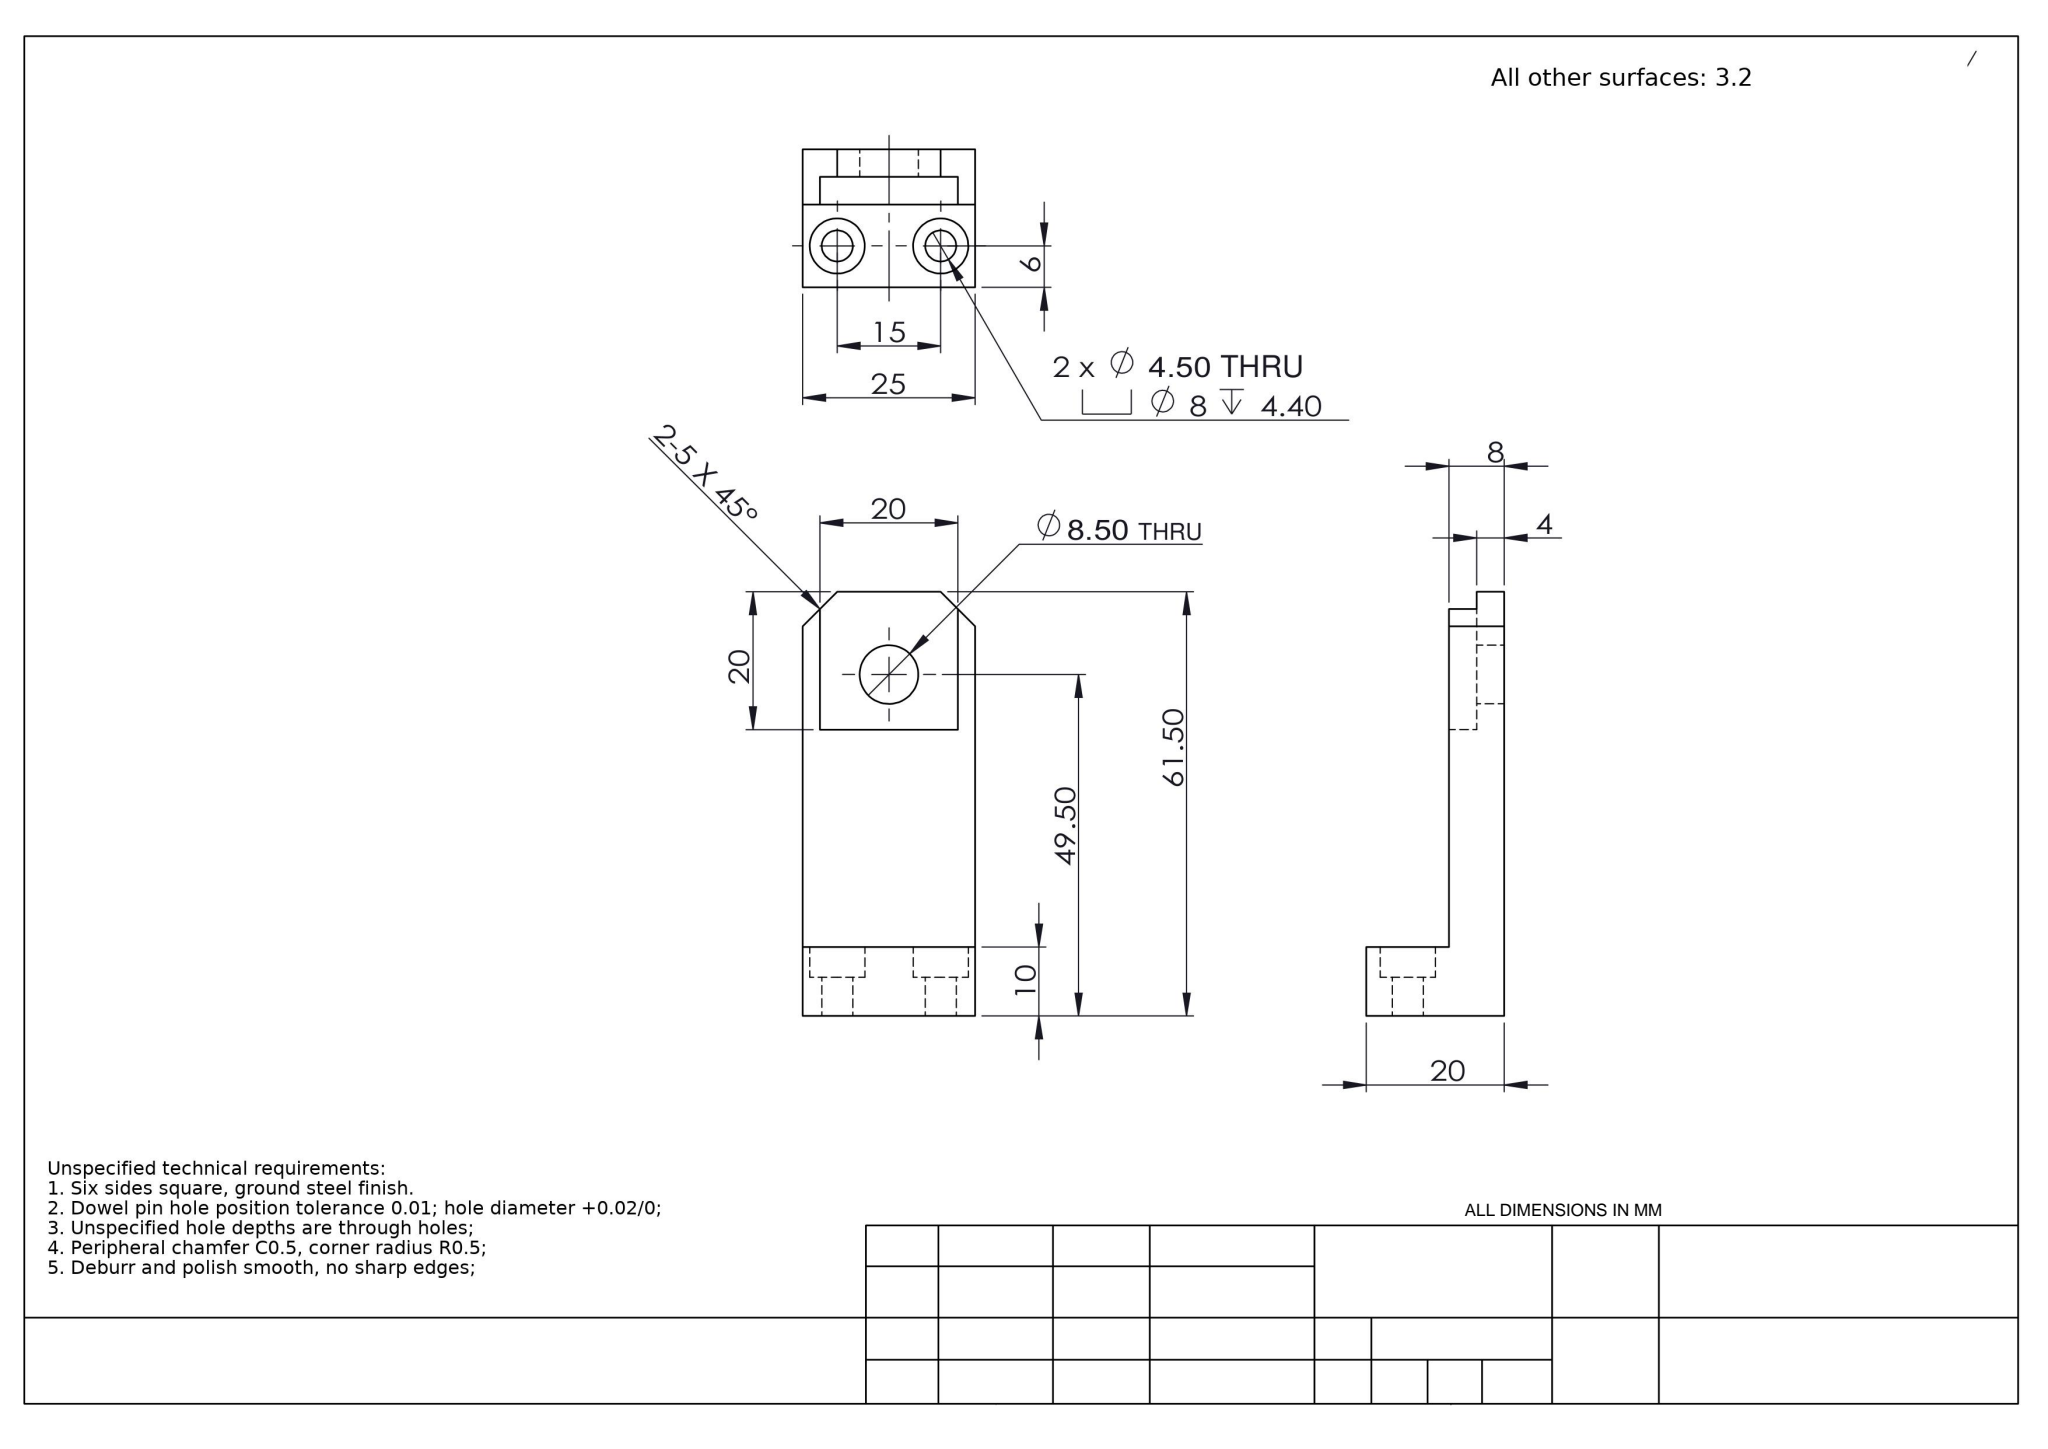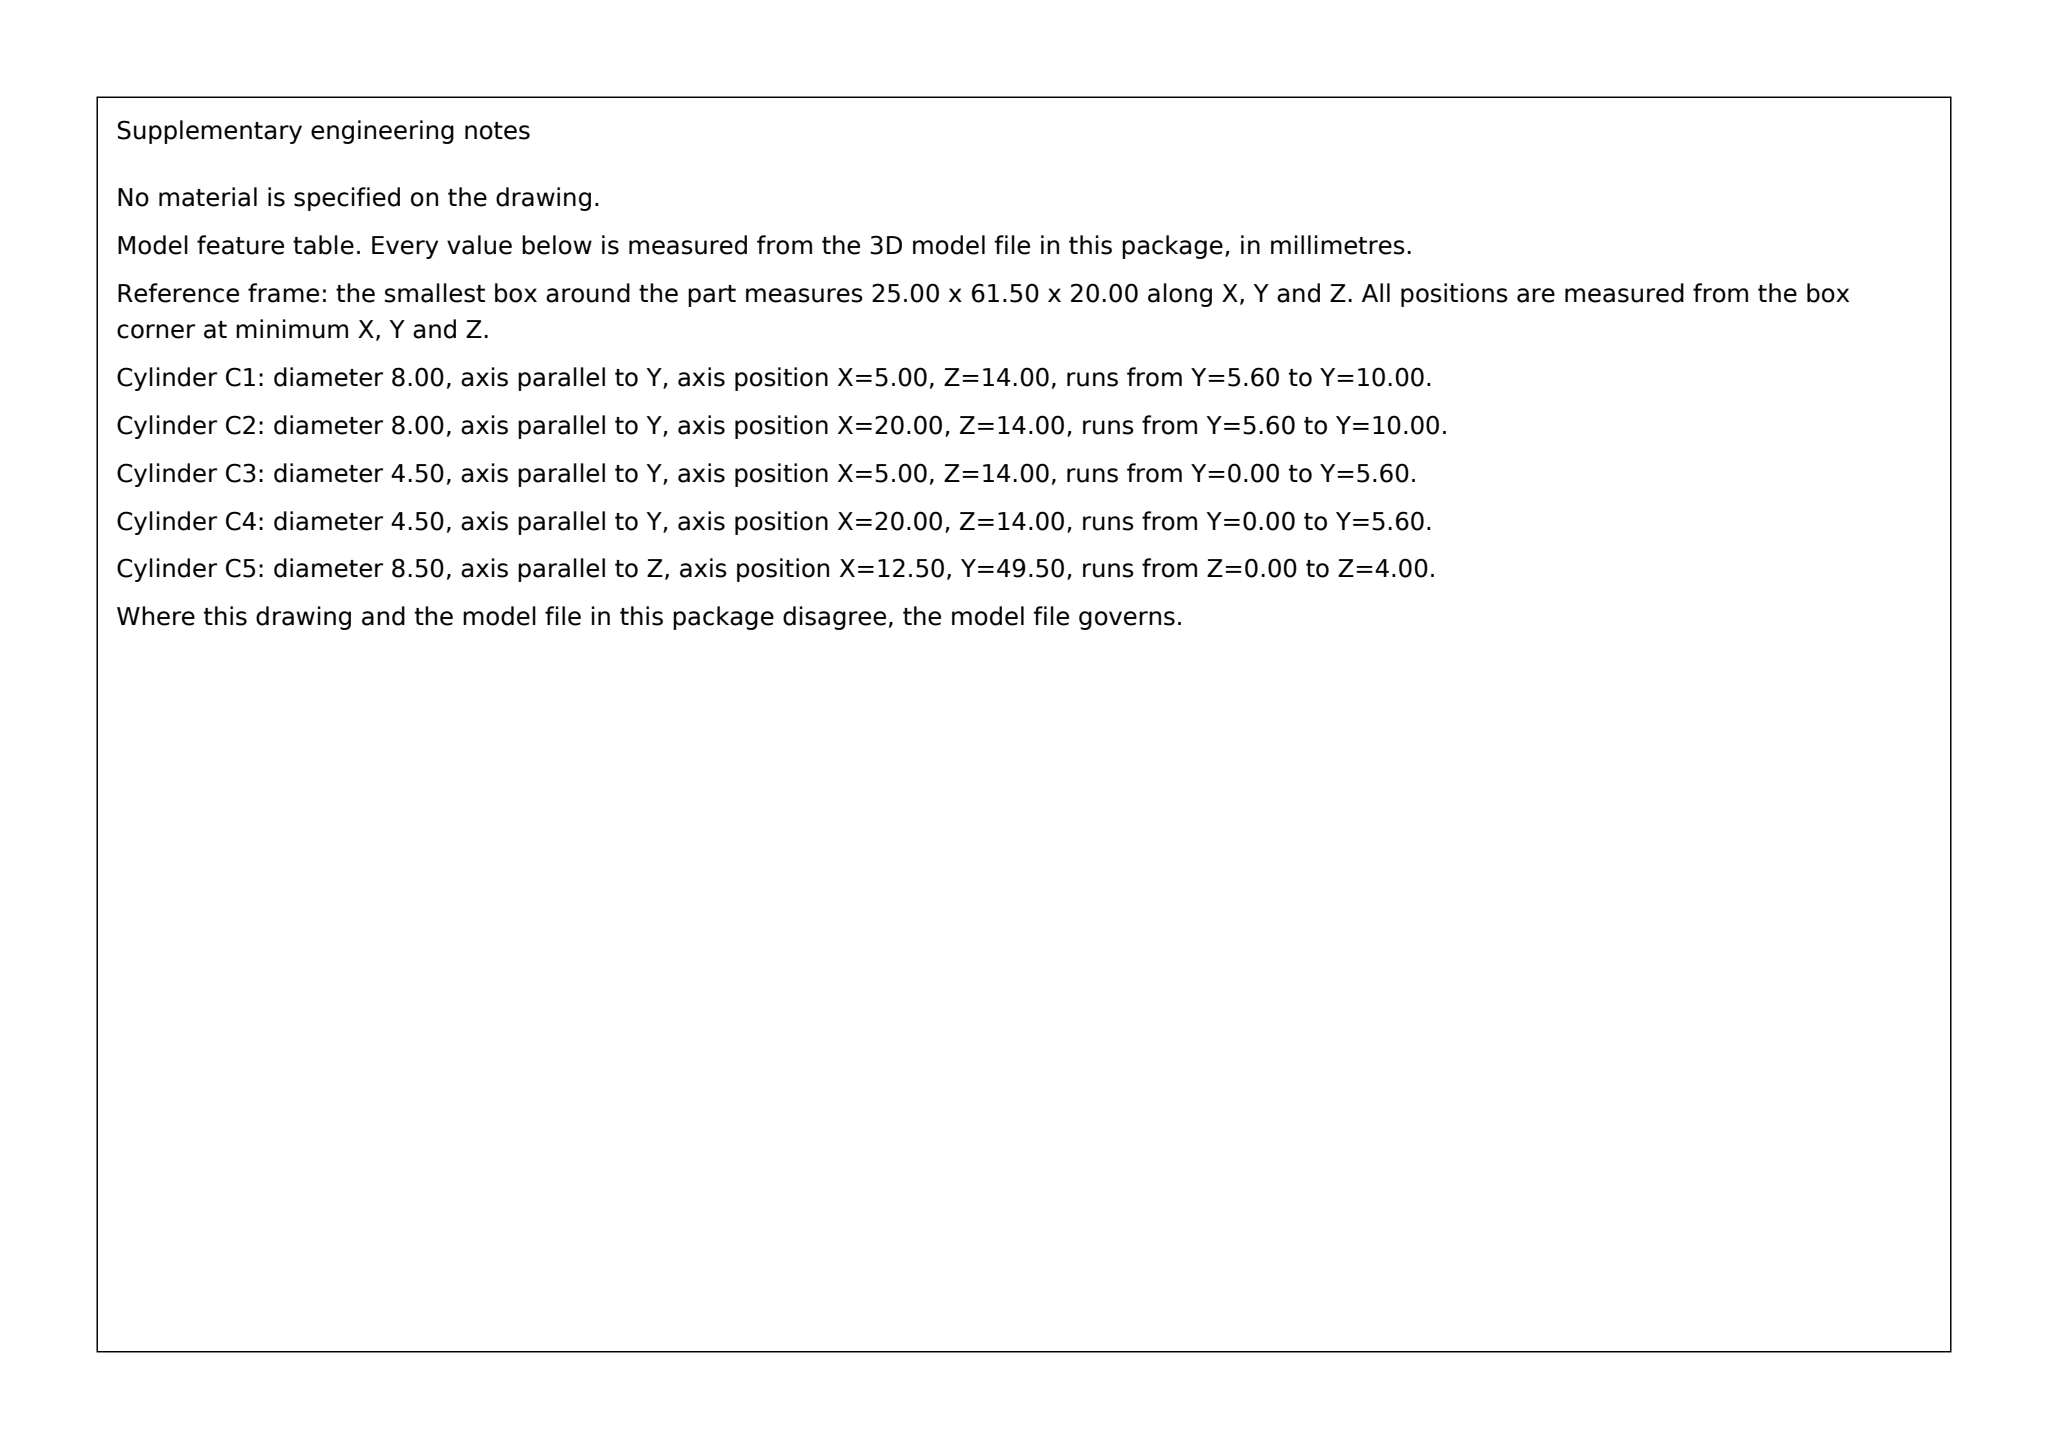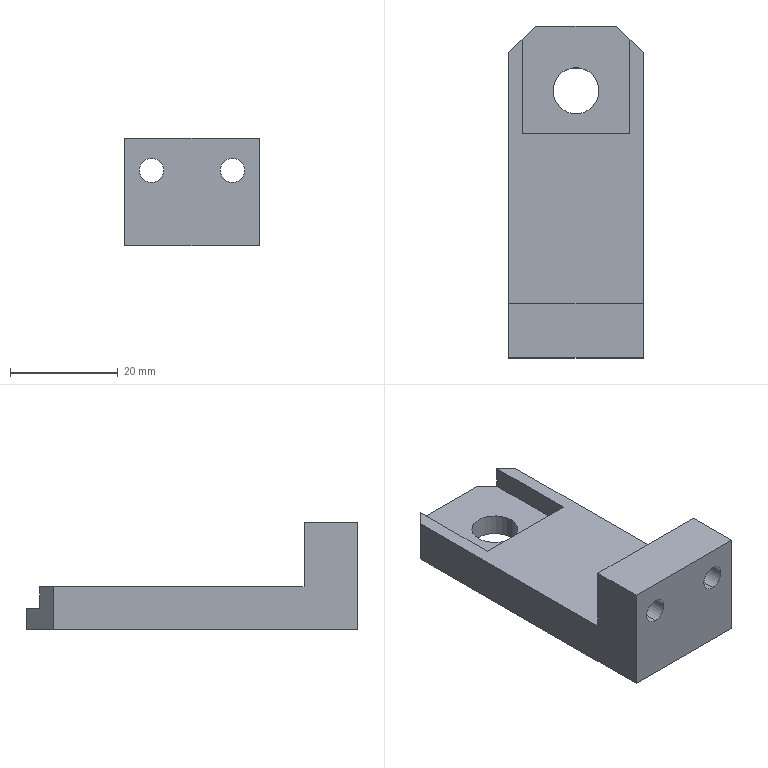Part | SolidWorks | mm | material 6060-T6 | 1 solid | 26 faces | box 25 x 61.5 x 20 mm | volume 12678 mm3 | plane 16 | cylinder 10 | commonest cylinder face diameters 8 x4 4.5 x4 8.5 x2
build123d program:
from build123d import *

# Parameters (mm, degrees)
SKETCH1_W                                       = 25
SKETCH1_H                                       = 20
BOSS_EXTRUDE1_DEPTH                             = 61.5
SKETCH2_W                                       = 12
SKETCH2_H                                       = 51.5
CUT_EXTRUDE1_DEPTH                              = 68.136
SKETCH3_R                                       = 4.25
CUT_EXTRUDE2_DEPTH                              = 64.894
M4_HEX_SOCKET_HEAD_CAP_SCREW_CBORE1_D           = 4.5
M4_HEX_SOCKET_HEAD_CAP_SCREW_CBORE1_CBORE_D     = 8
M4_HEX_SOCKET_HEAD_CAP_SCREW_CBORE1_CBORE_DEPTH = 4.4
CHAMFER1_SIZE                                   = 5
SKETCH7_W                                       = 20
SKETCH7_H                                       = 20
CUT_EXTRUDE3_DEPTH                              = 4


with BuildPart() as part:
    # Sketch1 → Boss-Extrude1 (new body)
    with BuildSketch(Plane(origin=(0, 0, 0), x_dir=(1, 0, 0), z_dir=(0, 1, 0))):
        Rectangle(SKETCH1_W, SKETCH1_H)
    extrude(amount=BOSS_EXTRUDE1_DEPTH)

    # Sketch2 → Cut-Extrude1 (cut, through all)
    with BuildSketch(Plane(origin=(12.5, 0, 0), x_dir=(0, 0, -1), z_dir=(1, 0, 0))):
        with Locations((-4, 35.75)):
            Rectangle(SKETCH2_W, SKETCH2_H)
    extrude(amount=-CUT_EXTRUDE1_DEPTH, mode=Mode.SUBTRACT)

    # Sketch3 → Cut-Extrude2 (cut, through all)
    with BuildSketch(Plane.XY.offset(-2)):
        with Locations((0, 49.5)):
            Circle(SKETCH3_R)
    extrude(amount=-CUT_EXTRUDE2_DEPTH, mode=Mode.SUBTRACT)

    # M4 Hex Socket Head Cap Screw CBORE1 (through all)
    with Locations(Plane(origin=(0, 10, 0), x_dir=(1, 0, 0), z_dir=(0, 1, 0))):
        with Locations((-7.5, -4), (7.5, -4)):
            CounterBoreHole(M4_HEX_SOCKET_HEAD_CAP_SCREW_CBORE1_D / 2, M4_HEX_SOCKET_HEAD_CAP_SCREW_CBORE1_CBORE_D / 2, M4_HEX_SOCKET_HEAD_CAP_SCREW_CBORE1_CBORE_DEPTH)

    # Chamfer1
    chamfer1_edges = [part.edges().sort_by_distance(p)[0] for p in [
        (-12.5, 61.5, -6),
        (12.5, 61.5, -6),
    ]]
    chamfer(chamfer1_edges, length=CHAMFER1_SIZE)

    # Sketch7 → Cut-Extrude3 (cut)
    with BuildSketch(Plane.XY.offset(-2)):
        with Locations((0, 51.5)):
            Rectangle(SKETCH7_W, SKETCH7_H)
    extrude(amount=-CUT_EXTRUDE3_DEPTH, mode=Mode.SUBTRACT)


solid = part.part
STEP:
#1=CARTESIAN_POINT('',(-7.5,5.6,-0.));
#2=VERTEX_POINT('',#1);
#3=CARTESIAN_POINT('',(-7.5,5.6,8.));
#4=VERTEX_POINT('',#3);
#5=CARTESIAN_POINT('',(-7.5,5.6,4.));
#6=DIRECTION('',(0.,1.,0.));
#7=DIRECTION('',(0.,0.,1.));
#8=AXIS2_PLACEMENT_3D('',#5,#6,#7);
#9=CIRCLE('',#8,4.);
#10=EDGE_CURVE('',#2,#4,#9,.T.);
#11=ORIENTED_EDGE('',*,*,#10,.F.);
#12=CARTESIAN_POINT('',(-7.5,10.,-0.));
#13=VERTEX_POINT('',#12);
#14=CARTESIAN_POINT('',(-7.5,10.,-0.));
#15=DIRECTION('',(0.,1.,0.));
#16=VECTOR('',#15,1000.);
#17=LINE('',#14,#16);
#18=EDGE_CURVE('',#2,#13,#17,.T.);
#19=ORIENTED_EDGE('',*,*,#18,.T.);
#20=CARTESIAN_POINT('',(-7.5,10.,8.));
#21=VERTEX_POINT('',#20);
#22=CARTESIAN_POINT('',(-7.5,10.,4.));
#23=DIRECTION('',(0.,1.,0.));
#24=DIRECTION('',(0.,0.,1.));
#25=AXIS2_PLACEMENT_3D('',#22,#23,#24);
#26=CIRCLE('',#25,4.);
#27=EDGE_CURVE('',#13,#21,#26,.T.);
#28=ORIENTED_EDGE('',*,*,#27,.T.);
#29=CARTESIAN_POINT('',(-7.5,10.,8.));
#30=DIRECTION('',(0.,1.,0.));
#31=VECTOR('',#30,1000.);
#32=LINE('',#29,#31);
#33=EDGE_CURVE('',#4,#21,#32,.T.);
#34=ORIENTED_EDGE('',*,*,#33,.F.);
#35=EDGE_LOOP('',(#11,#19,#28,#34));
#36=FACE_OUTER_BOUND('',#35,.T.);
#37=CARTESIAN_POINT('',(-7.5,10.,4.));
#38=DIRECTION('',(0.,1.,0.));
#39=DIRECTION('',(0.,0.,1.));
#40=AXIS2_PLACEMENT_3D('',#37,#38,#39);
#41=CYLINDRICAL_SURFACE('',#40,4.);
#42=ADVANCED_FACE('',(#36),#41,.F.);
#43=CARTESIAN_POINT('',(-7.5,0.,1.75));
#44=VERTEX_POINT('',#43);
#45=CARTESIAN_POINT('',(-7.5,0.,6.25));
#46=VERTEX_POINT('',#45);
#47=CARTESIAN_POINT('',(-7.5,0.,4.));
#48=DIRECTION('',(0.,1.,0.));
#49=DIRECTION('',(0.,0.,1.));
#50=AXIS2_PLACEMENT_3D('',#47,#48,#49);
#51=CIRCLE('',#50,2.25);
#52=EDGE_CURVE('',#44,#46,#51,.T.);
#53=ORIENTED_EDGE('',*,*,#52,.F.);
#54=CARTESIAN_POINT('',(-7.5,5.6,1.75));
#55=VERTEX_POINT('',#54);
#56=CARTESIAN_POINT('',(-7.5,10.,1.75));
#57=DIRECTION('',(0.,1.,0.));
#58=VECTOR('',#57,1000.);
#59=LINE('',#56,#58);
#60=EDGE_CURVE('',#44,#55,#59,.T.);
#61=ORIENTED_EDGE('',*,*,#60,.T.);
#62=CARTESIAN_POINT('',(-7.5,5.6,6.25));
#63=VERTEX_POINT('',#62);
#64=CARTESIAN_POINT('',(-7.5,5.6,4.));
#65=DIRECTION('',(0.,1.,0.));
#66=DIRECTION('',(0.,0.,1.));
#67=AXIS2_PLACEMENT_3D('',#64,#65,#66);
#68=CIRCLE('',#67,2.25);
#69=EDGE_CURVE('',#55,#63,#68,.T.);
#70=ORIENTED_EDGE('',*,*,#69,.T.);
#71=CARTESIAN_POINT('',(-7.5,10.,6.25));
#72=DIRECTION('',(0.,1.,0.));
#73=VECTOR('',#72,1000.);
#74=LINE('',#71,#73);
#75=EDGE_CURVE('',#46,#63,#74,.T.);
#76=ORIENTED_EDGE('',*,*,#75,.F.);
#77=EDGE_LOOP('',(#53,#61,#70,#76));
#78=FACE_OUTER_BOUND('',#77,.T.);
#79=CARTESIAN_POINT('',(-7.5,10.,4.));
#80=DIRECTION('',(0.,1.,0.));
#81=DIRECTION('',(0.,0.,1.));
#82=AXIS2_PLACEMENT_3D('',#79,#80,#81);
#83=CYLINDRICAL_SURFACE('',#82,2.25);
#84=ADVANCED_FACE('',(#78),#83,.F.);
#85=CARTESIAN_POINT('',(7.5,5.6,-0.));
#86=VERTEX_POINT('',#85);
#87=CARTESIAN_POINT('',(7.5,5.6,8.));
#88=VERTEX_POINT('',#87);
#89=CARTESIAN_POINT('',(7.5,5.6,4.));
#90=DIRECTION('',(0.,1.,0.));
#91=DIRECTION('',(0.,0.,1.));
#92=AXIS2_PLACEMENT_3D('',#89,#90,#91);
#93=CIRCLE('',#92,4.);
#94=EDGE_CURVE('',#86,#88,#93,.T.);
#95=ORIENTED_EDGE('',*,*,#94,.F.);
#96=CARTESIAN_POINT('',(7.5,10.,-0.));
#97=VERTEX_POINT('',#96);
#98=CARTESIAN_POINT('',(7.5,10.,-0.));
#99=DIRECTION('',(0.,1.,0.));
#100=VECTOR('',#99,1000.);
#101=LINE('',#98,#100);
#102=EDGE_CURVE('',#86,#97,#101,.T.);
#103=ORIENTED_EDGE('',*,*,#102,.T.);
#104=CARTESIAN_POINT('',(7.5,10.,8.));
#105=VERTEX_POINT('',#104);
#106=CARTESIAN_POINT('',(7.5,10.,4.));
#107=DIRECTION('',(0.,1.,0.));
#108=DIRECTION('',(0.,0.,1.));
#109=AXIS2_PLACEMENT_3D('',#106,#107,#108);
#110=CIRCLE('',#109,4.);
#111=EDGE_CURVE('',#97,#105,#110,.T.);
#112=ORIENTED_EDGE('',*,*,#111,.T.);
#113=CARTESIAN_POINT('',(7.5,10.,8.));
#114=DIRECTION('',(0.,1.,0.));
#115=VECTOR('',#114,1000.);
#116=LINE('',#113,#115);
#117=EDGE_CURVE('',#88,#105,#116,.T.);
#118=ORIENTED_EDGE('',*,*,#117,.F.);
#119=EDGE_LOOP('',(#95,#103,#112,#118));
#120=FACE_OUTER_BOUND('',#119,.T.);
#121=CARTESIAN_POINT('',(7.5,10.,4.));
#122=DIRECTION('',(0.,1.,0.));
#123=DIRECTION('',(0.,0.,1.));
#124=AXIS2_PLACEMENT_3D('',#121,#122,#123);
#125=CYLINDRICAL_SURFACE('',#124,4.);
#126=ADVANCED_FACE('',(#120),#125,.F.);
#127=CARTESIAN_POINT('',(7.5,0.,1.75));
#128=VERTEX_POINT('',#127);
#129=CARTESIAN_POINT('',(7.5,0.,6.25));
#130=VERTEX_POINT('',#129);
#131=CARTESIAN_POINT('',(7.5,0.,4.));
#132=DIRECTION('',(0.,1.,0.));
#133=DIRECTION('',(0.,0.,1.));
#134=AXIS2_PLACEMENT_3D('',#131,#132,#133);
#135=CIRCLE('',#134,2.25);
#136=EDGE_CURVE('',#128,#130,#135,.T.);
#137=ORIENTED_EDGE('',*,*,#136,.F.);
#138=CARTESIAN_POINT('',(7.5,5.6,1.75));
#139=VERTEX_POINT('',#138);
#140=CARTESIAN_POINT('',(7.5,10.,1.75));
#141=DIRECTION('',(0.,1.,0.));
#142=VECTOR('',#141,1000.);
#143=LINE('',#140,#142);
#144=EDGE_CURVE('',#128,#139,#143,.T.);
#145=ORIENTED_EDGE('',*,*,#144,.T.);
#146=CARTESIAN_POINT('',(7.5,5.6,6.25));
#147=VERTEX_POINT('',#146);
#148=CARTESIAN_POINT('',(7.5,5.6,4.));
#149=DIRECTION('',(0.,1.,0.));
#150=DIRECTION('',(0.,0.,1.));
#151=AXIS2_PLACEMENT_3D('',#148,#149,#150);
#152=CIRCLE('',#151,2.25);
#153=EDGE_CURVE('',#139,#147,#152,.T.);
#154=ORIENTED_EDGE('',*,*,#153,.T.);
#155=CARTESIAN_POINT('',(7.5,10.,6.25));
#156=DIRECTION('',(0.,1.,0.));
#157=VECTOR('',#156,1000.);
#158=LINE('',#155,#157);
#159=EDGE_CURVE('',#130,#147,#158,.T.);
#160=ORIENTED_EDGE('',*,*,#159,.F.);
#161=EDGE_LOOP('',(#137,#145,#154,#160));
#162=FACE_OUTER_BOUND('',#161,.T.);
#163=CARTESIAN_POINT('',(7.5,10.,4.));
#164=DIRECTION('',(0.,1.,0.));
#165=DIRECTION('',(0.,0.,1.));
#166=AXIS2_PLACEMENT_3D('',#163,#164,#165);
#167=CYLINDRICAL_SURFACE('',#166,2.25);
#168=ADVANCED_FACE('',(#162),#167,.F.);
#169=CARTESIAN_POINT('',(-4.25,49.5,-10.));
#170=VERTEX_POINT('',#169);
#171=CARTESIAN_POINT('',(4.25,49.5,-10.));
#172=VERTEX_POINT('',#171);
#173=CARTESIAN_POINT('',(-0.,49.5,-10.));
#174=DIRECTION('',(0.,0.,1.));
#175=DIRECTION('',(1.,0.,0.));
#176=AXIS2_PLACEMENT_3D('',#173,#174,#175);
#177=CIRCLE('',#176,4.25);
#178=EDGE_CURVE('',#170,#172,#177,.T.);
#179=ORIENTED_EDGE('',*,*,#178,.F.);
#180=CARTESIAN_POINT('',(-4.25,49.5,-6.));
#181=VERTEX_POINT('',#180);
#182=CARTESIAN_POINT('',(-4.25,49.5,-10.));
#183=DIRECTION('',(0.,0.,1.));
#184=VECTOR('',#183,1000.);
#185=LINE('',#182,#184);
#186=EDGE_CURVE('',#170,#181,#185,.T.);
#187=ORIENTED_EDGE('',*,*,#186,.T.);
#188=CARTESIAN_POINT('',(4.25,49.5,-6.));
#189=VERTEX_POINT('',#188);
#190=CARTESIAN_POINT('',(-0.,49.5,-6.));
#191=DIRECTION('',(0.,0.,1.));
#192=DIRECTION('',(-1.,0.,0.));
#193=AXIS2_PLACEMENT_3D('',#190,#191,#192);
#194=CIRCLE('',#193,4.25);
#195=EDGE_CURVE('',#181,#189,#194,.T.);
#196=ORIENTED_EDGE('',*,*,#195,.T.);
#197=CARTESIAN_POINT('',(4.25,49.5,-10.));
#198=DIRECTION('',(0.,0.,1.));
#199=VECTOR('',#198,1000.);
#200=LINE('',#197,#199);
#201=EDGE_CURVE('',#172,#189,#200,.T.);
#202=ORIENTED_EDGE('',*,*,#201,.F.);
#203=EDGE_LOOP('',(#179,#187,#196,#202));
#204=FACE_OUTER_BOUND('',#203,.T.);
#205=CARTESIAN_POINT('',(-0.,49.5,-10.));
#206=DIRECTION('',(0.,0.,1.));
#207=DIRECTION('',(1.,0.,0.));
#208=AXIS2_PLACEMENT_3D('',#205,#206,#207);
#209=CYLINDRICAL_SURFACE('',#208,4.25);
#210=ADVANCED_FACE('',(#204),#209,.F.);
#211=CARTESIAN_POINT('',(12.5,56.5,-10.));
#212=VERTEX_POINT('',#211);
#213=CARTESIAN_POINT('',(12.5,0.,-10.));
#214=VERTEX_POINT('',#213);
#215=CARTESIAN_POINT('',(12.5,61.5,-10.));
#216=DIRECTION('',(0.,-1.,0.));
#217=VECTOR('',#216,1000.);
#218=LINE('',#215,#217);
#219=EDGE_CURVE('',#212,#214,#218,.T.);
#220=ORIENTED_EDGE('',*,*,#219,.F.);
#221=CARTESIAN_POINT('',(12.5,56.5,-2.));
#222=VERTEX_POINT('',#221);
#223=CARTESIAN_POINT('',(12.5,56.5,-2.));
#224=DIRECTION('',(0.,0.,1.));
#225=VECTOR('',#224,1000.);
#226=LINE('',#223,#225);
#227=EDGE_CURVE('',#212,#222,#226,.T.);
#228=ORIENTED_EDGE('',*,*,#227,.T.);
#229=CARTESIAN_POINT('',(12.5,10.,-2.));
#230=VERTEX_POINT('',#229);
#231=CARTESIAN_POINT('',(12.5,61.5,-2.));
#232=DIRECTION('',(0.,1.,0.));
#233=VECTOR('',#232,1000.);
#234=LINE('',#231,#233);
#235=EDGE_CURVE('',#230,#222,#234,.T.);
#236=ORIENTED_EDGE('',*,*,#235,.F.);
#237=CARTESIAN_POINT('',(12.5,10.,10.));
#238=VERTEX_POINT('',#237);
#239=CARTESIAN_POINT('',(12.5,10.,10.));
#240=DIRECTION('',(-0.,-0.,-1.));
#241=VECTOR('',#240,1000.);
#242=LINE('',#239,#241);
#243=EDGE_CURVE('',#238,#230,#242,.T.);
#244=ORIENTED_EDGE('',*,*,#243,.F.);
#245=CARTESIAN_POINT('',(12.5,0.,10.));
#246=VERTEX_POINT('',#245);
#247=CARTESIAN_POINT('',(12.5,61.5,10.));
#248=DIRECTION('',(0.,-1.,0.));
#249=VECTOR('',#248,1000.);
#250=LINE('',#247,#249);
#251=EDGE_CURVE('',#238,#246,#250,.T.);
#252=ORIENTED_EDGE('',*,*,#251,.T.);
#253=CARTESIAN_POINT('',(12.5,0.,-10.));
#254=DIRECTION('',(-0.,0.,-1.));
#255=VECTOR('',#254,1000.);
#256=LINE('',#253,#255);
#257=EDGE_CURVE('',#246,#214,#256,.T.);
#258=ORIENTED_EDGE('',*,*,#257,.T.);
#259=EDGE_LOOP('',(#220,#228,#236,#244,#252,#258));
#260=FACE_OUTER_BOUND('',#259,.T.);
#261=CARTESIAN_POINT('',(12.5,61.5,-10.));
#262=DIRECTION('',(-1.,0.,0.));
#263=DIRECTION('',(0.,0.,1.));
#264=AXIS2_PLACEMENT_3D('',#261,#262,#263);
#265=PLANE('',#264);
#266=ADVANCED_FACE('',(#260),#265,.F.);
#267=CARTESIAN_POINT('',(-0.,49.5,-10.));
#268=DIRECTION('',(0.,0.,1.));
#269=DIRECTION('',(1.,0.,0.));
#270=AXIS2_PLACEMENT_3D('',#267,#268,#269);
#271=CIRCLE('',#270,4.25);
#272=EDGE_CURVE('',#172,#170,#271,.T.);
#273=ORIENTED_EDGE('',*,*,#272,.T.);
#274=ORIENTED_EDGE('',*,*,#178,.T.);
#275=EDGE_LOOP('',(#273,#274));
#276=FACE_BOUND('',#275,.T.);
#277=CARTESIAN_POINT('',(-12.5,56.5,-10.));
#278=VERTEX_POINT('',#277);
#279=CARTESIAN_POINT('',(-12.5,0.,-10.));
#280=VERTEX_POINT('',#279);
#281=CARTESIAN_POINT('',(-12.5,61.5,-10.));
#282=DIRECTION('',(0.,-1.,0.));
#283=VECTOR('',#282,1000.);
#284=LINE('',#281,#283);
#285=EDGE_CURVE('',#278,#280,#284,.T.);
#286=ORIENTED_EDGE('',*,*,#285,.F.);
#287=CARTESIAN_POINT('',(-7.5,61.5,-10.));
#288=VERTEX_POINT('',#287);
#289=CARTESIAN_POINT('',(-7.5,61.5,-10.));
#290=DIRECTION('',(0.7071,0.7071,0.));
#291=VECTOR('',#290,1000.);
#292=LINE('',#289,#291);
#293=EDGE_CURVE('',#278,#288,#292,.T.);
#294=ORIENTED_EDGE('',*,*,#293,.T.);
#295=CARTESIAN_POINT('',(7.5,61.5,-10.));
#296=VERTEX_POINT('',#295);
#297=CARTESIAN_POINT('',(-12.5,61.5,-10.));
#298=DIRECTION('',(-1.,0.,0.));
#299=VECTOR('',#298,1000.);
#300=LINE('',#297,#299);
#301=EDGE_CURVE('',#296,#288,#300,.T.);
#302=ORIENTED_EDGE('',*,*,#301,.F.);
#303=CARTESIAN_POINT('',(7.5,61.5,-10.));
#304=DIRECTION('',(0.7071,-0.7071,0.));
#305=VECTOR('',#304,1000.);
#306=LINE('',#303,#305);
#307=EDGE_CURVE('',#296,#212,#306,.T.);
#308=ORIENTED_EDGE('',*,*,#307,.T.);
#309=ORIENTED_EDGE('',*,*,#219,.T.);
#310=CARTESIAN_POINT('',(-12.5,0.,-10.));
#311=DIRECTION('',(-1.,0.,0.));
#312=VECTOR('',#311,1000.);
#313=LINE('',#310,#312);
#314=EDGE_CURVE('',#214,#280,#313,.T.);
#315=ORIENTED_EDGE('',*,*,#314,.T.);
#316=EDGE_LOOP('',(#286,#294,#302,#308,#309,#315));
#317=FACE_OUTER_BOUND('',#316,.T.);
#318=CARTESIAN_POINT('',(-12.5,61.5,-10.));
#319=DIRECTION('',(0.,0.,1.));
#320=DIRECTION('',(1.,0.,0.));
#321=AXIS2_PLACEMENT_3D('',#318,#319,#320);
#322=PLANE('',#321);
#323=ADVANCED_FACE('',(#276,#317),#322,.F.);
#324=CARTESIAN_POINT('',(-12.5,10.,-2.));
#325=VERTEX_POINT('',#324);
#326=CARTESIAN_POINT('',(-12.5,56.5,-2.));
#327=VERTEX_POINT('',#326);
#328=CARTESIAN_POINT('',(-12.5,61.5,-2.));
#329=DIRECTION('',(0.,1.,0.));
#330=VECTOR('',#329,1000.);
#331=LINE('',#328,#330);
#332=EDGE_CURVE('',#325,#327,#331,.T.);
#333=ORIENTED_EDGE('',*,*,#332,.T.);
#334=CARTESIAN_POINT('',(-12.5,56.5,-10.));
#335=DIRECTION('',(-0.,0.,-1.));
#336=VECTOR('',#335,1000.);
#337=LINE('',#334,#336);
#338=EDGE_CURVE('',#327,#278,#337,.T.);
#339=ORIENTED_EDGE('',*,*,#338,.T.);
#340=ORIENTED_EDGE('',*,*,#285,.T.);
#341=CARTESIAN_POINT('',(-12.5,0.,10.));
#342=VERTEX_POINT('',#341);
#343=CARTESIAN_POINT('',(-12.5,0.,-10.));
#344=DIRECTION('',(0.,0.,1.));
#345=VECTOR('',#344,1000.);
#346=LINE('',#343,#345);
#347=EDGE_CURVE('',#280,#342,#346,.T.);
#348=ORIENTED_EDGE('',*,*,#347,.T.);
#349=CARTESIAN_POINT('',(-12.5,10.,10.));
#350=VERTEX_POINT('',#349);
#351=CARTESIAN_POINT('',(-12.5,61.5,10.));
#352=DIRECTION('',(0.,-1.,0.));
#353=VECTOR('',#352,1000.);
#354=LINE('',#351,#353);
#355=EDGE_CURVE('',#350,#342,#354,.T.);
#356=ORIENTED_EDGE('',*,*,#355,.F.);
#357=CARTESIAN_POINT('',(-12.5,10.,10.));
#358=DIRECTION('',(-0.,-0.,-1.));
#359=VECTOR('',#358,1000.);
#360=LINE('',#357,#359);
#361=EDGE_CURVE('',#350,#325,#360,.T.);
#362=ORIENTED_EDGE('',*,*,#361,.T.);
#363=EDGE_LOOP('',(#333,#339,#340,#348,#356,#362));
#364=FACE_OUTER_BOUND('',#363,.T.);
#365=CARTESIAN_POINT('',(-12.5,61.5,-10.));
#366=DIRECTION('',(1.,0.,-0.));
#367=DIRECTION('',(-0.,0.,-1.));
#368=AXIS2_PLACEMENT_3D('',#365,#366,#367);
#369=PLANE('',#368);
#370=ADVANCED_FACE('',(#364),#369,.F.);
#371=ORIENTED_EDGE('',*,*,#251,.F.);
#372=CARTESIAN_POINT('',(-12.5,10.,10.));
#373=DIRECTION('',(1.,0.,-0.));
#374=VECTOR('',#373,1000.);
#375=LINE('',#372,#374);
#376=EDGE_CURVE('',#350,#238,#375,.T.);
#377=ORIENTED_EDGE('',*,*,#376,.F.);
#378=ORIENTED_EDGE('',*,*,#355,.T.);
#379=CARTESIAN_POINT('',(-12.5,0.,10.));
#380=DIRECTION('',(1.,0.,0.));
#381=VECTOR('',#380,1000.);
#382=LINE('',#379,#381);
#383=EDGE_CURVE('',#342,#246,#382,.T.);
#384=ORIENTED_EDGE('',*,*,#383,.T.);
#385=EDGE_LOOP('',(#371,#377,#378,#384));
#386=FACE_OUTER_BOUND('',#385,.T.);
#387=CARTESIAN_POINT('',(-12.5,61.5,10.));
#388=DIRECTION('',(0.,0.,-1.));
#389=DIRECTION('',(-1.,0.,0.));
#390=AXIS2_PLACEMENT_3D('',#387,#388,#389);
#391=PLANE('',#390);
#392=ADVANCED_FACE('',(#386),#391,.F.);
#393=CARTESIAN_POINT('',(7.5,61.5,-6.));
#394=VERTEX_POINT('',#393);
#395=CARTESIAN_POINT('',(-7.5,61.5,-6.));
#396=VERTEX_POINT('',#395);
#397=CARTESIAN_POINT('',(-10.,61.5,-6.));
#398=DIRECTION('',(-1.,0.,0.));
#399=VECTOR('',#398,1000.);
#400=LINE('',#397,#399);
#401=EDGE_CURVE('',#394,#396,#400,.T.);
#402=ORIENTED_EDGE('',*,*,#401,.F.);
#403=CARTESIAN_POINT('',(7.5,61.5,-10.));
#404=DIRECTION('',(-0.,0.,-1.));
#405=VECTOR('',#404,1000.);
#406=LINE('',#403,#405);
#407=EDGE_CURVE('',#394,#296,#406,.T.);
#408=ORIENTED_EDGE('',*,*,#407,.T.);
#409=ORIENTED_EDGE('',*,*,#301,.T.);
#410=CARTESIAN_POINT('',(-7.5,61.5,-2.));
#411=DIRECTION('',(0.,0.,1.));
#412=VECTOR('',#411,1000.);
#413=LINE('',#410,#412);
#414=EDGE_CURVE('',#288,#396,#413,.T.);
#415=ORIENTED_EDGE('',*,*,#414,.T.);
#416=EDGE_LOOP('',(#402,#408,#409,#415));
#417=FACE_OUTER_BOUND('',#416,.T.);
#418=CARTESIAN_POINT('',(0.,61.5,0.));
#419=DIRECTION('',(0.,1.,0.));
#420=DIRECTION('',(0.,0.,1.));
#421=AXIS2_PLACEMENT_3D('',#418,#419,#420);
#422=PLANE('',#421);
#423=ADVANCED_FACE('',(#417),#422,.T.);
#424=CARTESIAN_POINT('',(-7.5,0.,4.));
#425=DIRECTION('',(0.,1.,0.));
#426=DIRECTION('',(0.,0.,1.));
#427=AXIS2_PLACEMENT_3D('',#424,#425,#426);
#428=CIRCLE('',#427,2.25);
#429=EDGE_CURVE('',#46,#44,#428,.T.);
#430=ORIENTED_EDGE('',*,*,#429,.T.);
#431=ORIENTED_EDGE('',*,*,#52,.T.);
#432=EDGE_LOOP('',(#430,#431));
#433=FACE_BOUND('',#432,.T.);
#434=CARTESIAN_POINT('',(7.5,0.,4.));
#435=DIRECTION('',(0.,1.,0.));
#436=DIRECTION('',(0.,0.,1.));
#437=AXIS2_PLACEMENT_3D('',#434,#435,#436);
#438=CIRCLE('',#437,2.25);
#439=EDGE_CURVE('',#130,#128,#438,.T.);
#440=ORIENTED_EDGE('',*,*,#439,.T.);
#441=ORIENTED_EDGE('',*,*,#136,.T.);
#442=EDGE_LOOP('',(#440,#441));
#443=FACE_BOUND('',#442,.T.);
#444=ORIENTED_EDGE('',*,*,#257,.F.);
#445=ORIENTED_EDGE('',*,*,#383,.F.);
#446=ORIENTED_EDGE('',*,*,#347,.F.);
#447=ORIENTED_EDGE('',*,*,#314,.F.);
#448=EDGE_LOOP('',(#444,#445,#446,#447));
#449=FACE_OUTER_BOUND('',#448,.T.);
#450=CARTESIAN_POINT('',(0.,0.,0.));
#451=DIRECTION('',(0.,1.,0.));
#452=DIRECTION('',(0.,0.,1.));
#453=AXIS2_PLACEMENT_3D('',#450,#451,#452);
#454=PLANE('',#453);
#455=ADVANCED_FACE('',(#433,#443,#449),#454,.F.);
#456=CARTESIAN_POINT('',(-10.,41.5,-2.));
#457=VERTEX_POINT('',#456);
#458=CARTESIAN_POINT('',(10.,41.5,-2.));
#459=VERTEX_POINT('',#458);
#460=CARTESIAN_POINT('',(-10.,41.5,-2.));
#461=DIRECTION('',(1.,0.,0.));
#462=VECTOR('',#461,1000.);
#463=LINE('',#460,#462);
#464=EDGE_CURVE('',#457,#459,#463,.T.);
#465=ORIENTED_EDGE('',*,*,#464,.F.);
#466=CARTESIAN_POINT('',(-10.,59.,-2.));
#467=VERTEX_POINT('',#466);
#468=CARTESIAN_POINT('',(-10.,41.5,-2.));
#469=DIRECTION('',(0.,-1.,0.));
#470=VECTOR('',#469,1000.);
#471=LINE('',#468,#470);
#472=EDGE_CURVE('',#467,#457,#471,.T.);
#473=ORIENTED_EDGE('',*,*,#472,.F.);
#474=CARTESIAN_POINT('',(-7.5,61.5,-2.));
#475=DIRECTION('',(-0.7071,-0.7071,-0.));
#476=VECTOR('',#475,1000.);
#477=LINE('',#474,#476);
#478=EDGE_CURVE('',#467,#327,#477,.T.);
#479=ORIENTED_EDGE('',*,*,#478,.T.);
#480=ORIENTED_EDGE('',*,*,#332,.F.);
#481=CARTESIAN_POINT('',(-12.5,10.,-2.));
#482=DIRECTION('',(1.,0.,-0.));
#483=VECTOR('',#482,1000.);
#484=LINE('',#481,#483);
#485=EDGE_CURVE('',#325,#230,#484,.T.);
#486=ORIENTED_EDGE('',*,*,#485,.T.);
#487=ORIENTED_EDGE('',*,*,#235,.T.);
#488=CARTESIAN_POINT('',(10.,59.,-2.));
#489=VERTEX_POINT('',#488);
#490=CARTESIAN_POINT('',(7.5,61.5,-2.));
#491=DIRECTION('',(-0.7071,0.7071,0.));
#492=VECTOR('',#491,1000.);
#493=LINE('',#490,#492);
#494=EDGE_CURVE('',#222,#489,#493,.T.);
#495=ORIENTED_EDGE('',*,*,#494,.T.);
#496=CARTESIAN_POINT('',(10.,41.5,-2.));
#497=DIRECTION('',(-0.,1.,0.));
#498=VECTOR('',#497,1000.);
#499=LINE('',#496,#498);
#500=EDGE_CURVE('',#459,#489,#499,.T.);
#501=ORIENTED_EDGE('',*,*,#500,.F.);
#502=EDGE_LOOP('',(#465,#473,#479,#480,#486,#487,#495,#501));
#503=FACE_OUTER_BOUND('',#502,.T.);
#504=CARTESIAN_POINT('',(-12.5,61.5,-2.));
#505=DIRECTION('',(-0.,0.,-1.));
#506=DIRECTION('',(0.,1.,0.));
#507=AXIS2_PLACEMENT_3D('',#504,#505,#506);
#508=PLANE('',#507);
#509=ADVANCED_FACE('',(#503),#508,.F.);
#510=CARTESIAN_POINT('',(-7.5,10.,4.));
#511=DIRECTION('',(0.,1.,0.));
#512=DIRECTION('',(0.,0.,1.));
#513=AXIS2_PLACEMENT_3D('',#510,#511,#512);
#514=CIRCLE('',#513,4.);
#515=EDGE_CURVE('',#21,#13,#514,.T.);
#516=ORIENTED_EDGE('',*,*,#515,.F.);
#517=ORIENTED_EDGE('',*,*,#27,.F.);
#518=EDGE_LOOP('',(#516,#517));
#519=FACE_BOUND('',#518,.T.);
#520=CARTESIAN_POINT('',(7.5,10.,4.));
#521=DIRECTION('',(0.,1.,0.));
#522=DIRECTION('',(0.,0.,1.));
#523=AXIS2_PLACEMENT_3D('',#520,#521,#522);
#524=CIRCLE('',#523,4.);
#525=EDGE_CURVE('',#105,#97,#524,.T.);
#526=ORIENTED_EDGE('',*,*,#525,.F.);
#527=ORIENTED_EDGE('',*,*,#111,.F.);
#528=EDGE_LOOP('',(#526,#527));
#529=FACE_BOUND('',#528,.T.);
#530=ORIENTED_EDGE('',*,*,#243,.T.);
#531=ORIENTED_EDGE('',*,*,#485,.F.);
#532=ORIENTED_EDGE('',*,*,#361,.F.);
#533=ORIENTED_EDGE('',*,*,#376,.T.);
#534=EDGE_LOOP('',(#530,#531,#532,#533));
#535=FACE_OUTER_BOUND('',#534,.T.);
#536=CARTESIAN_POINT('',(-12.5,10.,10.));
#537=DIRECTION('',(0.,-1.,0.));
#538=DIRECTION('',(0.,-0.,-1.));
#539=AXIS2_PLACEMENT_3D('',#536,#537,#538);
#540=PLANE('',#539);
#541=ADVANCED_FACE('',(#519,#529,#535),#540,.F.);
#542=ORIENTED_EDGE('',*,*,#186,.F.);
#543=ORIENTED_EDGE('',*,*,#272,.F.);
#544=ORIENTED_EDGE('',*,*,#201,.T.);
#545=CARTESIAN_POINT('',(-0.,49.5,-6.));
#546=DIRECTION('',(0.,0.,1.));
#547=DIRECTION('',(-1.,0.,0.));
#548=AXIS2_PLACEMENT_3D('',#545,#546,#547);
#549=CIRCLE('',#548,4.25);
#550=EDGE_CURVE('',#189,#181,#549,.T.);
#551=ORIENTED_EDGE('',*,*,#550,.T.);
#552=EDGE_LOOP('',(#542,#543,#544,#551));
#553=FACE_OUTER_BOUND('',#552,.T.);
#554=CARTESIAN_POINT('',(-0.,49.5,-10.));
#555=DIRECTION('',(0.,0.,1.));
#556=DIRECTION('',(1.,0.,0.));
#557=AXIS2_PLACEMENT_3D('',#554,#555,#556);
#558=CYLINDRICAL_SURFACE('',#557,4.25);
#559=ADVANCED_FACE('',(#553),#558,.F.);
#560=ORIENTED_EDGE('',*,*,#144,.F.);
#561=ORIENTED_EDGE('',*,*,#439,.F.);
#562=ORIENTED_EDGE('',*,*,#159,.T.);
#563=CARTESIAN_POINT('',(7.5,5.6,4.));
#564=DIRECTION('',(0.,1.,0.));
#565=DIRECTION('',(0.,0.,1.));
#566=AXIS2_PLACEMENT_3D('',#563,#564,#565);
#567=CIRCLE('',#566,2.25);
#568=EDGE_CURVE('',#147,#139,#567,.T.);
#569=ORIENTED_EDGE('',*,*,#568,.T.);
#570=EDGE_LOOP('',(#560,#561,#562,#569));
#571=FACE_OUTER_BOUND('',#570,.T.);
#572=CARTESIAN_POINT('',(7.5,10.,4.));
#573=DIRECTION('',(0.,1.,0.));
#574=DIRECTION('',(0.,0.,1.));
#575=AXIS2_PLACEMENT_3D('',#572,#573,#574);
#576=CYLINDRICAL_SURFACE('',#575,2.25);
#577=ADVANCED_FACE('',(#571),#576,.F.);
#578=ORIENTED_EDGE('',*,*,#568,.F.);
#579=ORIENTED_EDGE('',*,*,#153,.F.);
#580=EDGE_LOOP('',(#578,#579));
#581=FACE_BOUND('',#580,.T.);
#582=CARTESIAN_POINT('',(7.5,5.6,4.));
#583=DIRECTION('',(0.,1.,0.));
#584=DIRECTION('',(0.,0.,1.));
#585=AXIS2_PLACEMENT_3D('',#582,#583,#584);
#586=CIRCLE('',#585,4.);
#587=EDGE_CURVE('',#88,#86,#586,.T.);
#588=ORIENTED_EDGE('',*,*,#587,.T.);
#589=ORIENTED_EDGE('',*,*,#94,.T.);
#590=EDGE_LOOP('',(#588,#589));
#591=FACE_OUTER_BOUND('',#590,.T.);
#592=CARTESIAN_POINT('',(9.75,5.6,4.));
#593=DIRECTION('',(0.,-1.,0.));
#594=DIRECTION('',(0.,0.,-1.));
#595=AXIS2_PLACEMENT_3D('',#592,#593,#594);
#596=PLANE('',#595);
#597=ADVANCED_FACE('',(#581,#591),#596,.F.);
#598=ORIENTED_EDGE('',*,*,#102,.F.);
#599=ORIENTED_EDGE('',*,*,#587,.F.);
#600=ORIENTED_EDGE('',*,*,#117,.T.);
#601=ORIENTED_EDGE('',*,*,#525,.T.);
#602=EDGE_LOOP('',(#598,#599,#600,#601));
#603=FACE_OUTER_BOUND('',#602,.T.);
#604=CARTESIAN_POINT('',(7.5,10.,4.));
#605=DIRECTION('',(0.,1.,0.));
#606=DIRECTION('',(0.,0.,1.));
#607=AXIS2_PLACEMENT_3D('',#604,#605,#606);
#608=CYLINDRICAL_SURFACE('',#607,4.);
#609=ADVANCED_FACE('',(#603),#608,.F.);
#610=ORIENTED_EDGE('',*,*,#60,.F.);
#611=ORIENTED_EDGE('',*,*,#429,.F.);
#612=ORIENTED_EDGE('',*,*,#75,.T.);
#613=CARTESIAN_POINT('',(-7.5,5.6,4.));
#614=DIRECTION('',(0.,1.,0.));
#615=DIRECTION('',(0.,0.,1.));
#616=AXIS2_PLACEMENT_3D('',#613,#614,#615);
#617=CIRCLE('',#616,2.25);
#618=EDGE_CURVE('',#63,#55,#617,.T.);
#619=ORIENTED_EDGE('',*,*,#618,.T.);
#620=EDGE_LOOP('',(#610,#611,#612,#619));
#621=FACE_OUTER_BOUND('',#620,.T.);
#622=CARTESIAN_POINT('',(-7.5,10.,4.));
#623=DIRECTION('',(0.,1.,0.));
#624=DIRECTION('',(0.,0.,1.));
#625=AXIS2_PLACEMENT_3D('',#622,#623,#624);
#626=CYLINDRICAL_SURFACE('',#625,2.25);
#627=ADVANCED_FACE('',(#621),#626,.F.);
#628=ORIENTED_EDGE('',*,*,#618,.F.);
#629=ORIENTED_EDGE('',*,*,#69,.F.);
#630=EDGE_LOOP('',(#628,#629));
#631=FACE_BOUND('',#630,.T.);
#632=CARTESIAN_POINT('',(-7.5,5.6,4.));
#633=DIRECTION('',(0.,1.,0.));
#634=DIRECTION('',(0.,0.,1.));
#635=AXIS2_PLACEMENT_3D('',#632,#633,#634);
#636=CIRCLE('',#635,4.);
#637=EDGE_CURVE('',#4,#2,#636,.T.);
#638=ORIENTED_EDGE('',*,*,#637,.T.);
#639=ORIENTED_EDGE('',*,*,#10,.T.);
#640=EDGE_LOOP('',(#638,#639));
#641=FACE_OUTER_BOUND('',#640,.T.);
#642=CARTESIAN_POINT('',(-5.25,5.6,4.));
#643=DIRECTION('',(0.,-1.,0.));
#644=DIRECTION('',(0.,0.,-1.));
#645=AXIS2_PLACEMENT_3D('',#642,#643,#644);
#646=PLANE('',#645);
#647=ADVANCED_FACE('',(#631,#641),#646,.F.);
#648=ORIENTED_EDGE('',*,*,#18,.F.);
#649=ORIENTED_EDGE('',*,*,#637,.F.);
#650=ORIENTED_EDGE('',*,*,#33,.T.);
#651=ORIENTED_EDGE('',*,*,#515,.T.);
#652=EDGE_LOOP('',(#648,#649,#650,#651));
#653=FACE_OUTER_BOUND('',#652,.T.);
#654=CARTESIAN_POINT('',(-7.5,10.,4.));
#655=DIRECTION('',(0.,1.,0.));
#656=DIRECTION('',(0.,0.,1.));
#657=AXIS2_PLACEMENT_3D('',#654,#655,#656);
#658=CYLINDRICAL_SURFACE('',#657,4.);
#659=ADVANCED_FACE('',(#653),#658,.F.);
#660=CARTESIAN_POINT('',(-10.,59.,-6.));
#661=VERTEX_POINT('',#660);
#662=CARTESIAN_POINT('',(-10.,59.,0.));
#663=DIRECTION('',(0.,-0.,1.));
#664=VECTOR('',#663,1000.);
#665=LINE('',#662,#664);
#666=EDGE_CURVE('',#661,#467,#665,.T.);
#667=ORIENTED_EDGE('',*,*,#666,.F.);
#668=CARTESIAN_POINT('',(-7.5,61.5,-6.));
#669=DIRECTION('',(-0.7071,-0.7071,0.));
#670=VECTOR('',#669,1000.);
#671=LINE('',#668,#670);
#672=EDGE_CURVE('',#396,#661,#671,.T.);
#673=ORIENTED_EDGE('',*,*,#672,.F.);
#674=ORIENTED_EDGE('',*,*,#414,.F.);
#675=ORIENTED_EDGE('',*,*,#293,.F.);
#676=ORIENTED_EDGE('',*,*,#338,.F.);
#677=ORIENTED_EDGE('',*,*,#478,.F.);
#678=EDGE_LOOP('',(#667,#673,#674,#675,#676,#677));
#679=FACE_OUTER_BOUND('',#678,.T.);
#680=CARTESIAN_POINT('',(-7.5,61.5,0.));
#681=DIRECTION('',(-0.7071,0.7071,0.));
#682=DIRECTION('',(-0.,0.,-1.));
#683=AXIS2_PLACEMENT_3D('',#680,#681,#682);
#684=PLANE('',#683);
#685=ADVANCED_FACE('',(#679),#684,.T.);
#686=CARTESIAN_POINT('',(10.,59.,-6.));
#687=VERTEX_POINT('',#686);
#688=CARTESIAN_POINT('',(10.,59.,-0.));
#689=DIRECTION('',(0.,-0.,-1.));
#690=VECTOR('',#689,1000.);
#691=LINE('',#688,#690);
#692=EDGE_CURVE('',#489,#687,#691,.T.);
#693=ORIENTED_EDGE('',*,*,#692,.F.);
#694=ORIENTED_EDGE('',*,*,#494,.F.);
#695=ORIENTED_EDGE('',*,*,#227,.F.);
#696=ORIENTED_EDGE('',*,*,#307,.F.);
#697=ORIENTED_EDGE('',*,*,#407,.F.);
#698=CARTESIAN_POINT('',(7.5,61.5,-6.));
#699=DIRECTION('',(-0.7071,0.7071,0.));
#700=VECTOR('',#699,1000.);
#701=LINE('',#698,#700);
#702=EDGE_CURVE('',#687,#394,#701,.T.);
#703=ORIENTED_EDGE('',*,*,#702,.F.);
#704=EDGE_LOOP('',(#693,#694,#695,#696,#697,#703));
#705=FACE_OUTER_BOUND('',#704,.T.);
#706=CARTESIAN_POINT('',(7.5,61.5,-0.));
#707=DIRECTION('',(0.7071,0.7071,-0.));
#708=DIRECTION('',(0.,0.,1.));
#709=AXIS2_PLACEMENT_3D('',#706,#707,#708);
#710=PLANE('',#709);
#711=ADVANCED_FACE('',(#705),#710,.T.);
#712=ORIENTED_EDGE('',*,*,#672,.T.);
#713=CARTESIAN_POINT('',(-10.,41.5,-6.));
#714=VERTEX_POINT('',#713);
#715=CARTESIAN_POINT('',(-10.,41.5,-6.));
#716=DIRECTION('',(0.,-1.,0.));
#717=VECTOR('',#716,1000.);
#718=LINE('',#715,#717);
#719=EDGE_CURVE('',#661,#714,#718,.T.);
#720=ORIENTED_EDGE('',*,*,#719,.T.);
#721=CARTESIAN_POINT('',(10.,41.5,-6.));
#722=VERTEX_POINT('',#721);
#723=CARTESIAN_POINT('',(-10.,41.5,-6.));
#724=DIRECTION('',(1.,0.,0.));
#725=VECTOR('',#724,1000.);
#726=LINE('',#723,#725);
#727=EDGE_CURVE('',#714,#722,#726,.T.);
#728=ORIENTED_EDGE('',*,*,#727,.T.);
#729=CARTESIAN_POINT('',(10.,41.5,-6.));
#730=DIRECTION('',(-0.,1.,0.));
#731=VECTOR('',#730,1000.);
#732=LINE('',#729,#731);
#733=EDGE_CURVE('',#722,#687,#732,.T.);
#734=ORIENTED_EDGE('',*,*,#733,.T.);
#735=ORIENTED_EDGE('',*,*,#702,.T.);
#736=ORIENTED_EDGE('',*,*,#401,.T.);
#737=EDGE_LOOP('',(#712,#720,#728,#734,#735,#736));
#738=FACE_OUTER_BOUND('',#737,.T.);
#739=ORIENTED_EDGE('',*,*,#550,.F.);
#740=ORIENTED_EDGE('',*,*,#195,.F.);
#741=EDGE_LOOP('',(#739,#740));
#742=FACE_BOUND('',#741,.T.);
#743=CARTESIAN_POINT('',(0.,0.,-6.));
#744=DIRECTION('',(0.,0.,-1.));
#745=DIRECTION('',(-1.,0.,0.));
#746=AXIS2_PLACEMENT_3D('',#743,#744,#745);
#747=PLANE('',#746);
#748=ADVANCED_FACE('',(#738,#742),#747,.F.);
#749=ORIENTED_EDGE('',*,*,#666,.T.);
#750=ORIENTED_EDGE('',*,*,#472,.T.);
#751=CARTESIAN_POINT('',(-10.,41.5,-6.));
#752=DIRECTION('',(0.,0.,1.));
#753=VECTOR('',#752,1000.);
#754=LINE('',#751,#753);
#755=EDGE_CURVE('',#714,#457,#754,.T.);
#756=ORIENTED_EDGE('',*,*,#755,.F.);
#757=ORIENTED_EDGE('',*,*,#719,.F.);
#758=EDGE_LOOP('',(#749,#750,#756,#757));
#759=FACE_OUTER_BOUND('',#758,.T.);
#760=CARTESIAN_POINT('',(-10.,41.5,-6.));
#761=DIRECTION('',(-1.,-0.,0.));
#762=DIRECTION('',(0.,-1.,0.));
#763=AXIS2_PLACEMENT_3D('',#760,#761,#762);
#764=PLANE('',#763);
#765=ADVANCED_FACE('',(#759),#764,.F.);
#766=ORIENTED_EDGE('',*,*,#692,.T.);
#767=ORIENTED_EDGE('',*,*,#733,.F.);
#768=CARTESIAN_POINT('',(10.,41.5,-6.));
#769=DIRECTION('',(0.,0.,1.));
#770=VECTOR('',#769,1000.);
#771=LINE('',#768,#770);
#772=EDGE_CURVE('',#722,#459,#771,.T.);
#773=ORIENTED_EDGE('',*,*,#772,.T.);
#774=ORIENTED_EDGE('',*,*,#500,.T.);
#775=EDGE_LOOP('',(#766,#767,#773,#774));
#776=FACE_OUTER_BOUND('',#775,.T.);
#777=CARTESIAN_POINT('',(10.,41.5,-6.));
#778=DIRECTION('',(1.,0.,0.));
#779=DIRECTION('',(-0.,1.,0.));
#780=AXIS2_PLACEMENT_3D('',#777,#778,#779);
#781=PLANE('',#780);
#782=ADVANCED_FACE('',(#776),#781,.F.);
#783=ORIENTED_EDGE('',*,*,#464,.T.);
#784=ORIENTED_EDGE('',*,*,#772,.F.);
#785=ORIENTED_EDGE('',*,*,#727,.F.);
#786=ORIENTED_EDGE('',*,*,#755,.T.);
#787=EDGE_LOOP('',(#783,#784,#785,#786));
#788=FACE_OUTER_BOUND('',#787,.T.);
#789=CARTESIAN_POINT('',(-10.,41.5,-6.));
#790=DIRECTION('',(0.,-1.,0.));
#791=DIRECTION('',(0.,0.,-1.));
#792=AXIS2_PLACEMENT_3D('',#789,#790,#791);
#793=PLANE('',#792);
#794=ADVANCED_FACE('',(#788),#793,.F.);
#795=CLOSED_SHELL('',(#42,#84,#126,#168,#210,#266,#323,#370,#392,#423,#455,#509,#541,#559,#577,#597,#609,#627,#647,#659,#685,#711,#748,#765,#782,#794));
#796=MANIFOLD_SOLID_BREP('',#795);
#797=CARTESIAN_POINT('',(0.,0.,0.));
#798=DIRECTION('',(0.,0.,1.));
#799=DIRECTION('',(1.,0.,0.));
#800=AXIS2_PLACEMENT_3D('',#797,#798,#799);
#801=(LENGTH_UNIT()NAMED_UNIT(*)SI_UNIT(.MILLI.,.METRE.));
#802=UNCERTAINTY_MEASURE_WITH_UNIT(LENGTH_MEASURE(0.00001),#801,'','');
#803=(NAMED_UNIT(*)PLANE_ANGLE_UNIT()SI_UNIT($,.RADIAN.));
#804=(NAMED_UNIT(*)SI_UNIT($,.STERADIAN.)SOLID_ANGLE_UNIT());
#805=(GEOMETRIC_REPRESENTATION_CONTEXT(3)GLOBAL_UNCERTAINTY_ASSIGNED_CONTEXT((#802))GLOBAL_UNIT_ASSIGNED_CONTEXT((#801,#803,#804))REPRESENTATION_CONTEXT('',''));
#806=ADVANCED_BREP_SHAPE_REPRESENTATION('',(#796,#800),#805);